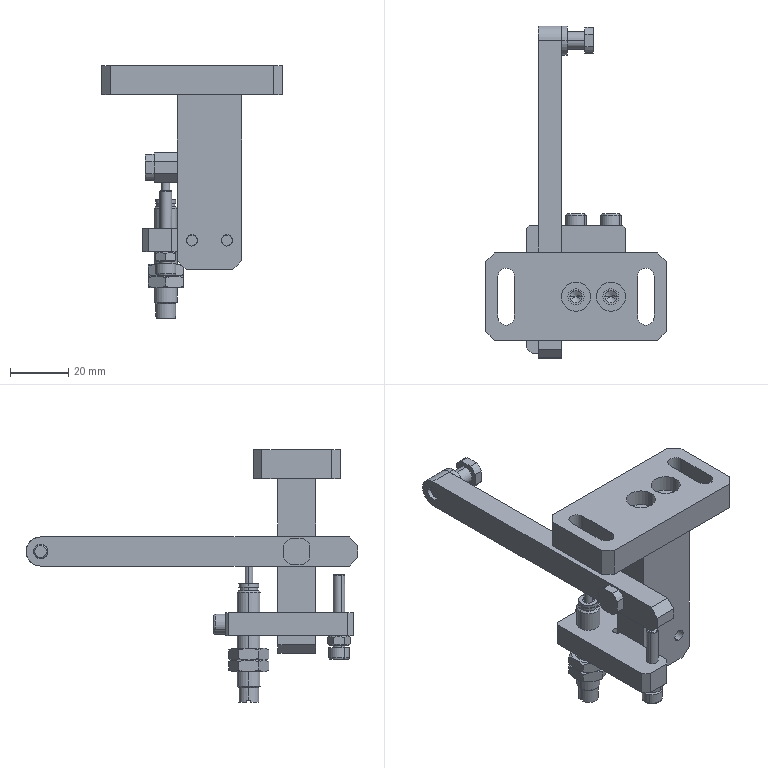Assembly | SolidWorks | mm | 14 component files | 14 solids | 306 faces | box 62 x 114 x 86.8 mm | volume 51199 mm3 | plane 143 | cylinder 91 | cone 64 | spline 8 | commonest cylinder face diameters 4 x20 10 x16 5 x8 6 x8 8 x8 7 x6 4.2 x4 6.8 x4
Bill of materials:
A47 | 1 | S136 | Tall rectangular block with cross-drilled holes and two chamfered corners at one end.
A48 | 1 | S136 | Long flat bar with a rectangular cross-section, a hole near each end, one rounded end and one end with chamfered corners.
A49 | 1 | S45C | Thick flat ring (annulus) with a plain central bore.
A50 | 1 | S45C | L-shaped flat plate with through holes, a round relief at the inside corner, cross holes in the inner edge and chamfered outer corners.
A51 | 2 | SUS304 | Stepped pin with an octagon-like flat-sided head, a larger cylindrical shank, a narrow groove, and a smaller cylindrical end with a chamfer.
A52 | 1 | A6061 | Rectangular flat plate with chamfered corners, two long slots near the ends and two round holes placed off-centre.
M4 | 1 | Standard Part | Hex nut-shaped part with chamfered corners on both faces and a countersunk round bore.
M4X25 | 3 | Standard Part | Cylindrical-headed pin or plain shank fastener: a short round head on a long plain cylindrical shank.
RB0806-1 | 1 |  | Stepped cylindrical shaft: a small-diameter spigot, a collar step, a long main body, and a smaller end section with a small notch at the far end.
RB0806-2 | 1 |  | Low-profile hex nut-shaped part with chamfered corners and a large chamfered round bore.
RB0806-3 | 1 |  | Low-profile hex nut-shaped part with chamfered corners and a large chamfered round bore.
Mates:
1. concentric | A47-1 face at (4.649, 25.864, 5) dir (1, 0, 0) r 2.5 | A48-1 face at (-17.351, 25.864, 5) dir (1, 0, 0) r 3
2. concentric | A48-1 face at (-17.351, 113.864, 5) dir (1, 0, 0) r 2.5 | A49-1 face at (-15.351, 113.864, 5) dir (-1, 0, 0) r 3
3. coincident | A48-1 face at (-17.351, 61.864, 5) dir (1, 0, 0) | A49-1 face at (-17.351, 113.864, 5) dir (-1, 0, 0)
4. parallel | A48-1 face at (-17.351, 4.864, 10) dir (0, 0, 1) | A49-1 plane at (-16.351, 113.864, 5) dir (0, 0, 1)
5. angle | A48-1 face at (-17.351, 4.864, 10) dir (0, 0, 1) | A47-1 face at (4.649, 32.364, 30) dir (0, 1, 0)
6. concentric | RB0806-1/RB0806-1-1 face at (-21.351, 42.364, -25.1) dir (0, 0, -1) r 4 | A50-1 face at (-21.351, 42.364, -16) dir (0, 0, 1) r 4
7. distance | RB0806-1/RB0806-1-1 face at (-21.351, 40.689, -6) dir (0, 0, 1) | A50-1 face at (-12.351, 41.364, -16) dir (0, 0, 1)
8. coincident | A47-1 face at (-17.351, 25.864, 0) dir (-1, 0, 0) | A48-1 face at (-17.351, 61.864, 5) dir (1, 0, 0)
9. parallel | A47-1 face at (-17.351, 25.864, 0) dir (-1, 0, 0) | A50-1 face at (-29.351, 32.364, -16) dir (-1, 0, 0)
10. distance | RB0806-1/RB0806-1-1 face at (-21.351, 42.364, 0) dir (0, 0, 1) | A47-1 face at (4.649, 32.364, 30) dir (0, 0, 1)
11. parallel | A48-1 face at (-25.351, 61.864, 5) dir (-1, 0, 0) | RB0806-1/RB0806-1-1 plane at (-21.351, 42.364, -6) dir (-1, 0, 0)
12. distance | RB0806-1/RB0806-1-1 plane at (-21.351, 42.364, -6) dir (-1, 0, 0) | A48-1 face at (-25.351, 61.864, 5) dir (-1, 0, 0)
13. coincident | A47-1 face at (4.649, 32.364, 30) dir (0, 1, 0) | A50-1 face at (4.649, 32.364, -16) dir (0, -1, 0)
14. concentric | A50-1 face at (-12.351, 50.364, -20) dir (0, 1, 0) r 2.25 | M4X25-2 face at (-12.351, 25.364, -20) dir (0, 1, 0) r 2
15. coincident | A50-1 face at (4.649, 50.364, -16) dir (0, 1, 0) | M4X25-2 face at (-12.351, 50.364, -20) dir (0, -1, 0)
16. parallel | A50-1 face at (4.649, 32.364, -16) dir (1, 0, 0) | M4X25-2 face at (-13.851, 52.364, -19.134) dir (1, 0, 0)
17. concentric | A50-1 face at (-0.3508, 50.364, -20) dir (0, 1, 0) r 2.25 | M4X25-3 face at (-0.3508, 25.364, -20) dir (0, 1, 0) r 2
18. coincident | A50-1 face at (4.649, 50.364, -16) dir (0, 1, 0) | M4X25-3 face at (-0.3508, 50.364, -20) dir (0, -1, 0)
19. parallel | A50-1 face at (4.649, 32.364, -16) dir (1, 0, 0) | M4X25-3 face at (-1.851, 52.364, -19.134) dir (1, 0, 0)
20. coincident | A47-1 face at (4.649, 32.364, 30) dir (0, 0, 1) | A52-1 face at (-12.351, 25.864, 30) dir (0, 0, -1)
21. width | A52-1 face at (-43.351, 40.864, 40) dir (0, 1, 0) | A52-1 face at (-43.351, 10.864, 40) dir (0, -1, 0) | A47-1 face at (4.649, 19.364, 30) dir (0, -1, 0) | A47-1 face at (4.649, 32.364, 30) dir (0, 1, 0)
22. concentric | A50-1 face at (-21.351, 11.364, -24) dir (0, 0, -1) r 2 | M4X25-5 face at (-21.351, 11.364, -3) dir (0, 0, -1) r 2
23. distance | A50-1 face at (-12.351, 41.364, -24) dir (0, 0, -1) | M4X25-5 face at (-21.351, 11.364, -28) dir (0, 0, 1)
24. coincident | A50-1 face at (-12.351, 41.364, -24) dir (0, 0, -1) | M4-3 face at (-17.851, 9.344, -24) dir (0, 0, 1)
25. concentric | M4X25-5 face at (-21.351, 11.364, -3) dir (0, 0, -1) r 2 | M4-3 face at (-21.351, 11.364, -27.2) dir (0, 0, 1) r 2
26. parallel | A50-1 face at (-29.351, 32.364, -16) dir (-1, 0, 0) | M4-3 face at (-24.851, 13.385, -27.2) dir (-1, 0, 0)
27. parallel | A50-1 face at (-29.351, 32.364, -16) dir (-1, 0, 0) | M4X25-5 face at (-19.851, 10.498, -30) dir (-1, 0, 0)
28. concentric | A48-1 face at (-17.351, 25.864, 5) dir (1, 0, 0) r 3 | A51-3 face at (-17.351, 25.864, 5) dir (-1, 0, 0) r 3
29. coincident | A48-1 face at (-25.351, 61.864, 5) dir (-1, 0, 0) | A51-3 face at (-25.351, 25.864, 5) dir (1, 0, 0)
30. parallel | A47-1 face at (4.649, 32.364, 30) dir (0, 1, 0) | A51-3 face at (-10.351, 30.364, 0.5) dir (0, 1, 0)
31. parallel | A48-1 face at (-17.351, 4.864, 0) dir (0, 0, -1) | A51-4 face at (-24.351, 118.364, 0.5) dir (0, 0, -1)
32. width | A47-1 face at (4.649, 25.864, 0) dir (1, 0, 0) | A50-1 face at (-29.351, 32.364, -16) dir (-1, 0, 0) | A52-1 face at (-43.351, 40.864, 40) dir (-1, 0, 0) | A52-1 face at (18.649, 40.864, 40) dir (1, 0, 0)